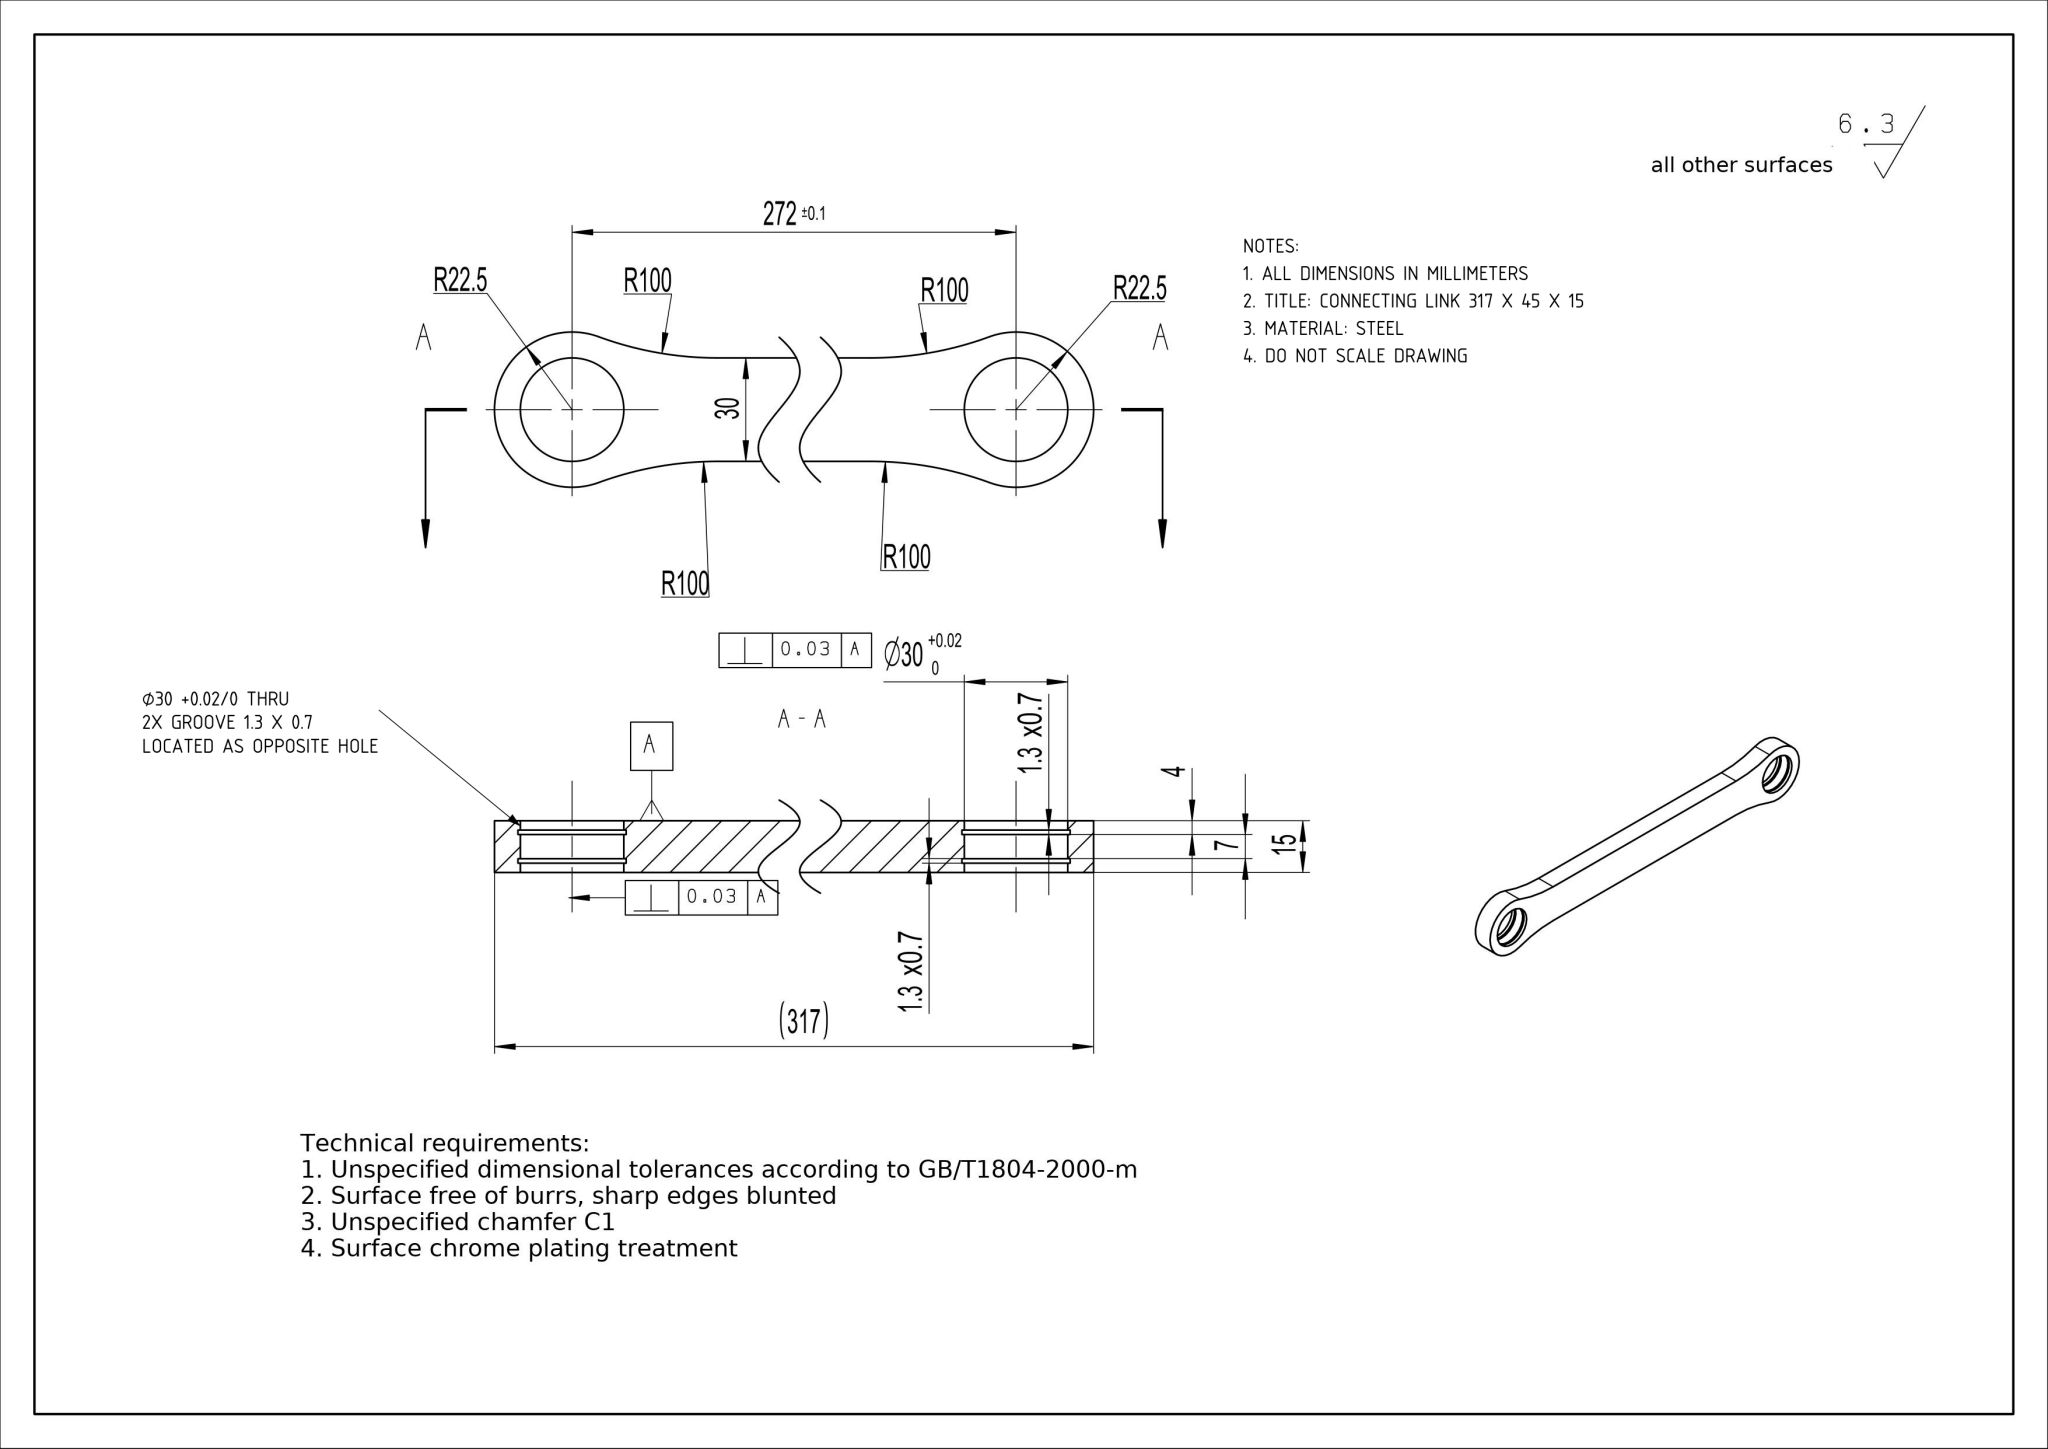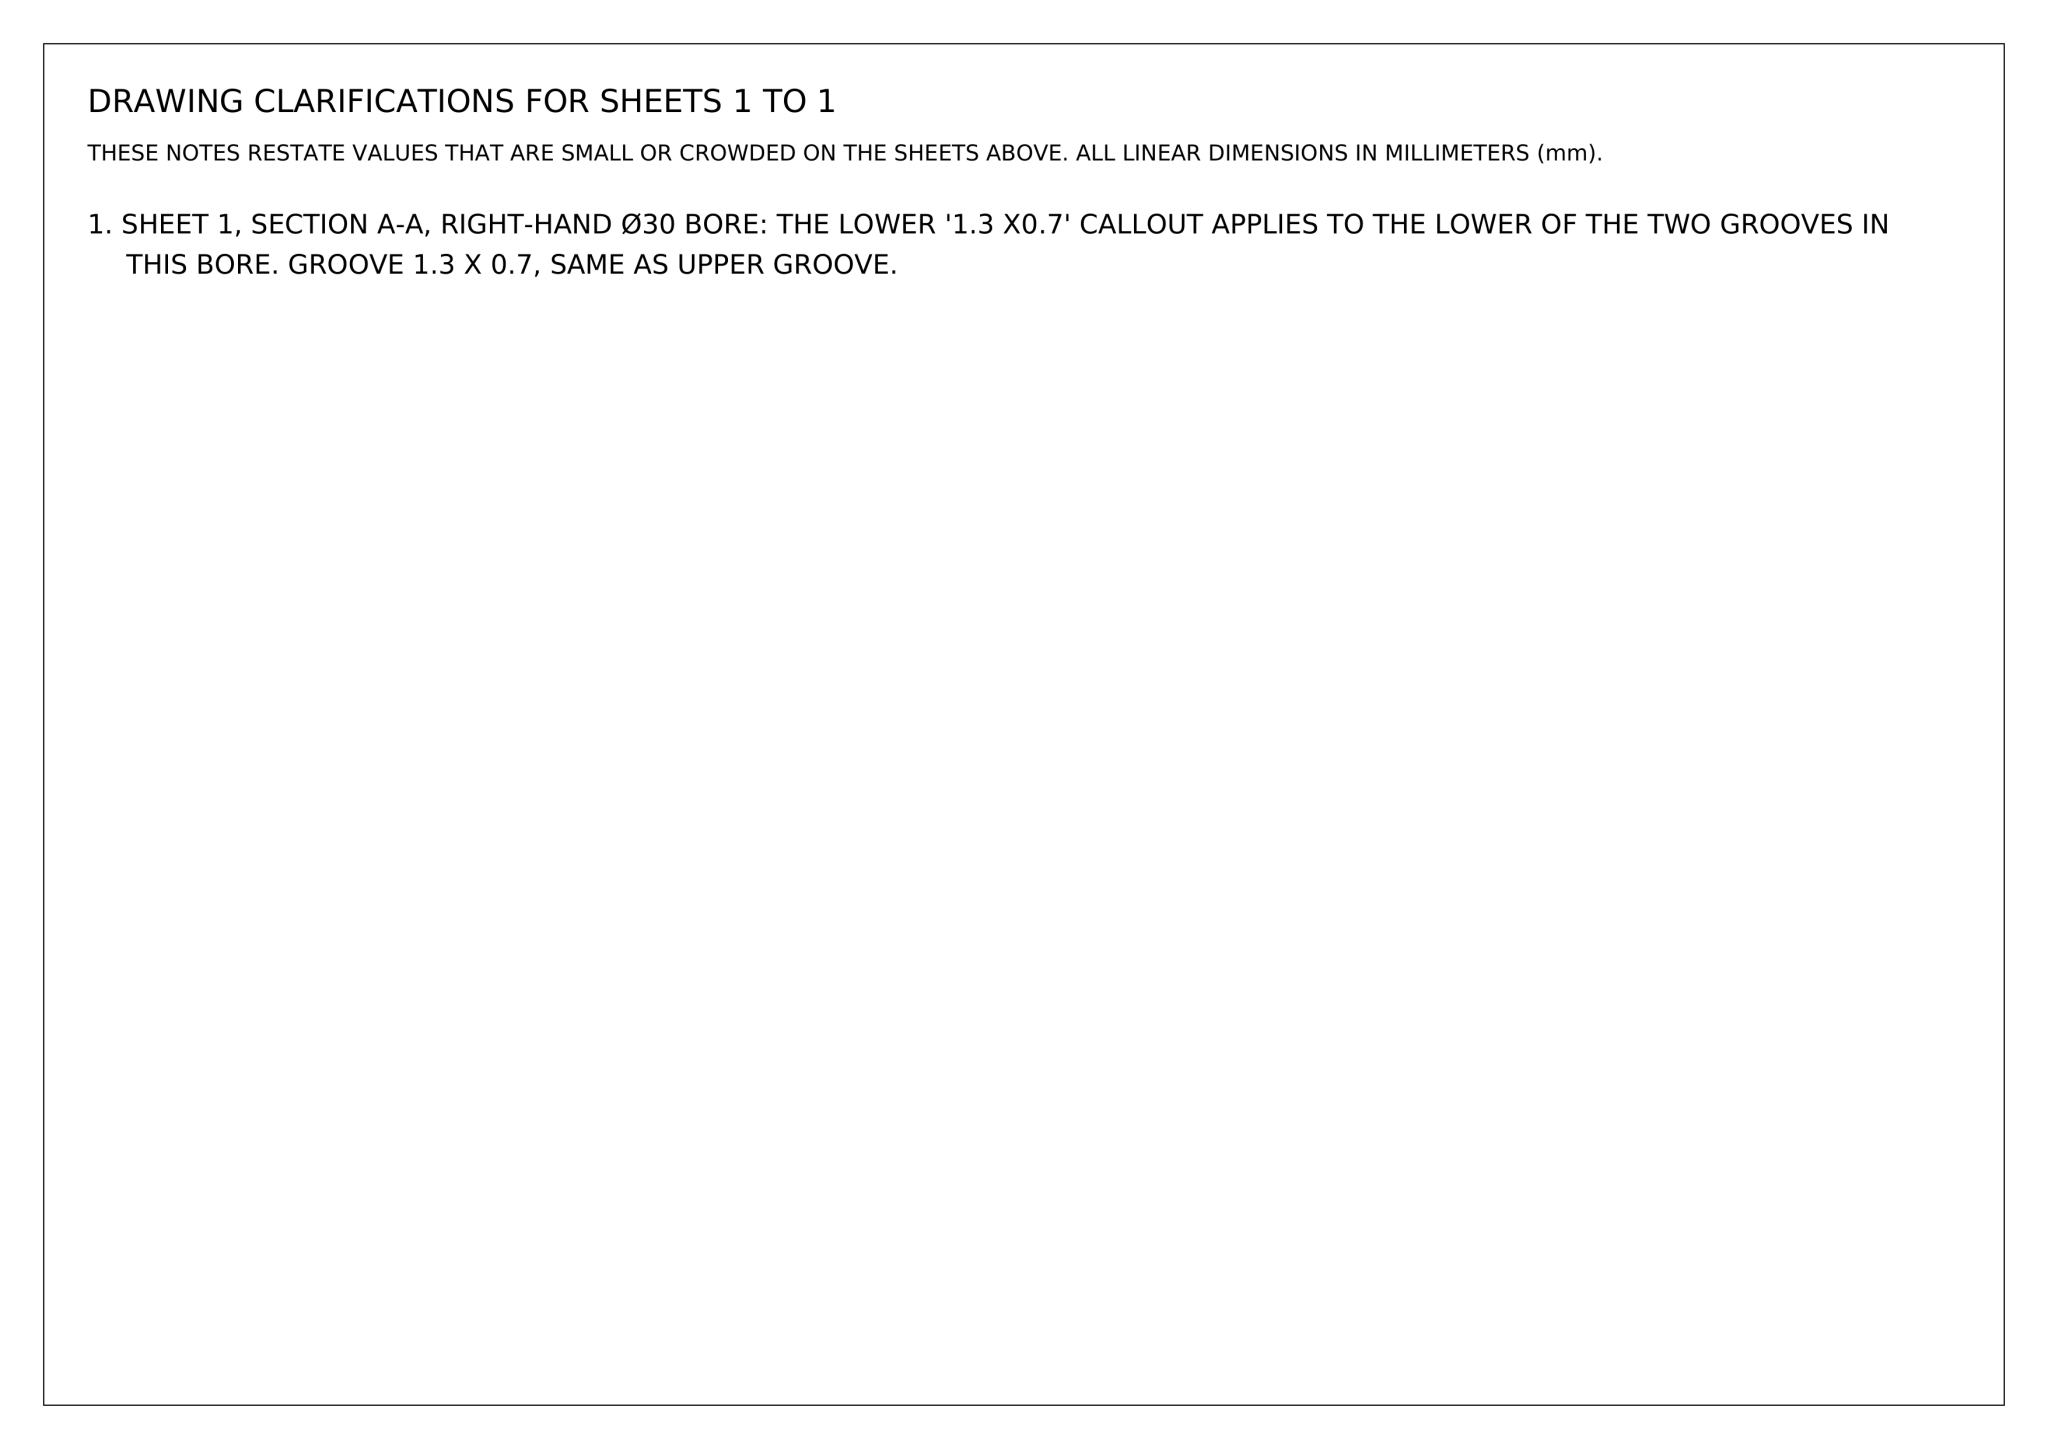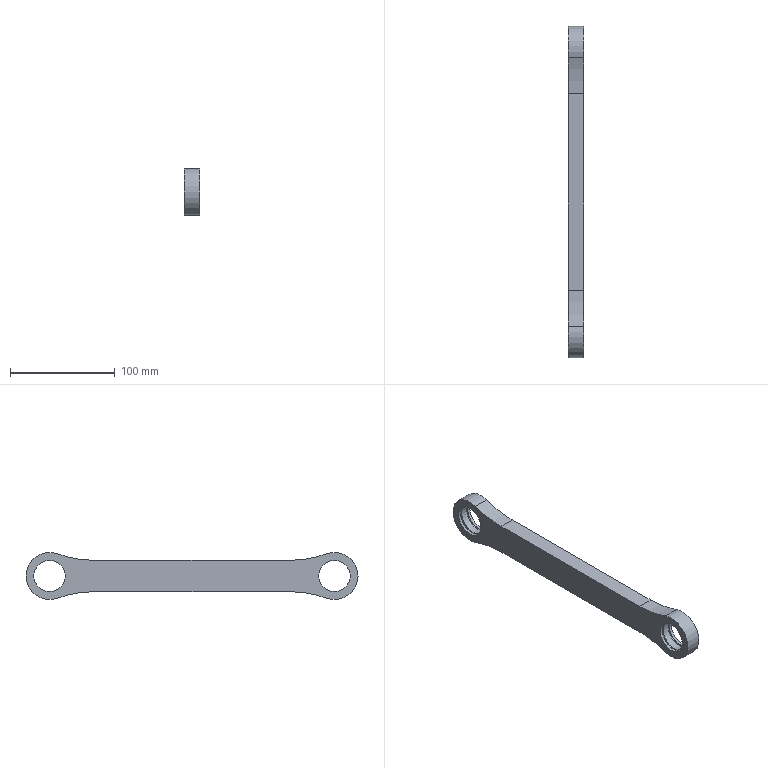Part | NX | mm | 1 solid | 28 faces | box 15 x 317 x 45 mm | volume 132143 mm3 | cylinder 16 | plane 12 | commonest cylinder face diameters 30 x6 31.4 x4 200 x4 45 x2
STEP:
#1=CARTESIAN_POINT('',(0.,0.,0.));
#2=DIRECTION('',(0.,0.,1.));
#3=DIRECTION('',(1.,0.,0.));
#4=AXIS2_PLACEMENT_3D('',#1,#2,#3);
#5=(LENGTH_UNIT()NAMED_UNIT(*)SI_UNIT(.MILLI.,.METRE.));
#6=UNCERTAINTY_MEASURE_WITH_UNIT(LENGTH_MEASURE(0.00002),#5,'','');
#7=(NAMED_UNIT(*)PLANE_ANGLE_UNIT()SI_UNIT($,.RADIAN.));
#8=PLANE_ANGLE_MEASURE_WITH_UNIT(PLANE_ANGLE_MEASURE(0.01745),#7);
#9=DIMENSIONAL_EXPONENTS(0.,0.,0.,0.,0.,0.,0.);
#10=(CONVERSION_BASED_UNIT('',#8)NAMED_UNIT(#9)PLANE_ANGLE_UNIT());
#11=(NAMED_UNIT(*)SI_UNIT($,.STERADIAN.)SOLID_ANGLE_UNIT());
#12=(GEOMETRIC_REPRESENTATION_CONTEXT(3)GLOBAL_UNCERTAINTY_ASSIGNED_CONTEXT((#6))GLOBAL_UNIT_ASSIGNED_CONTEXT((#5,#10,#11))REPRESENTATION_CONTEXT('',''));
#13=SHAPE_REPRESENTATION('',(#4),#12);
#14=CARTESIAN_POINT('',(4.,277.,-15.));
#15=VERTEX_POINT('',#14);
#16=CARTESIAN_POINT('',(4.,277.,0.));
#17=DIRECTION('',(1.,0.,0.));
#18=DIRECTION('',(0.,0.,-1.));
#19=AXIS2_PLACEMENT_3D('',#16,#17,#18);
#20=CIRCLE('',#19,15.);
#21=EDGE_CURVE('',#15,#15,#20,.T.);
#22=ORIENTED_EDGE('',*,*,#21,.F.);
#23=EDGE_LOOP('',(#22));
#24=FACE_BOUND('',#23,.T.);
#25=CARTESIAN_POINT('',(11.,277.,-15.));
#26=VERTEX_POINT('',#25);
#27=CARTESIAN_POINT('',(11.,277.,0.));
#28=DIRECTION('',(1.,0.,0.));
#29=DIRECTION('',(0.,0.,-1.));
#30=AXIS2_PLACEMENT_3D('',#27,#28,#29);
#31=CIRCLE('',#30,15.);
#32=EDGE_CURVE('',#26,#26,#31,.T.);
#33=ORIENTED_EDGE('',*,*,#32,.T.);
#34=EDGE_LOOP('',(#33));
#35=FACE_BOUND('',#34,.T.);
#36=CARTESIAN_POINT('',(15.,277.,0.));
#37=DIRECTION('',(-1.,0.,0.));
#38=DIRECTION('',(0.,0.,1.));
#39=AXIS2_PLACEMENT_3D('',#36,#37,#38);
#40=CYLINDRICAL_SURFACE('',#39,15.);
#41=ADVANCED_FACE('',(#24,#35),#40,.F.);
#42=CARTESIAN_POINT('',(0.,277.,-15.));
#43=VERTEX_POINT('',#42);
#44=CARTESIAN_POINT('',(0.,277.,0.));
#45=DIRECTION('',(1.,0.,0.));
#46=DIRECTION('',(0.,0.,-1.));
#47=AXIS2_PLACEMENT_3D('',#44,#45,#46);
#48=CIRCLE('',#47,15.);
#49=EDGE_CURVE('',#43,#43,#48,.T.);
#50=ORIENTED_EDGE('',*,*,#49,.F.);
#51=EDGE_LOOP('',(#50));
#52=FACE_BOUND('',#51,.T.);
#53=CARTESIAN_POINT('',(2.7,277.,-15.));
#54=VERTEX_POINT('',#53);
#55=CARTESIAN_POINT('',(2.7,277.,0.));
#56=DIRECTION('',(1.,0.,0.));
#57=DIRECTION('',(0.,0.,-1.));
#58=AXIS2_PLACEMENT_3D('',#55,#56,#57);
#59=CIRCLE('',#58,15.);
#60=EDGE_CURVE('',#54,#54,#59,.T.);
#61=ORIENTED_EDGE('',*,*,#60,.T.);
#62=EDGE_LOOP('',(#61));
#63=FACE_BOUND('',#62,.T.);
#64=CARTESIAN_POINT('',(15.,277.,0.));
#65=DIRECTION('',(-1.,0.,0.));
#66=DIRECTION('',(0.,0.,1.));
#67=AXIS2_PLACEMENT_3D('',#64,#65,#66);
#68=CYLINDRICAL_SURFACE('',#67,15.);
#69=ADVANCED_FACE('',(#52,#63),#68,.F.);
#70=CARTESIAN_POINT('',(4.,5.,-15.));
#71=VERTEX_POINT('',#70);
#72=CARTESIAN_POINT('',(4.,5.,0.));
#73=DIRECTION('',(1.,0.,0.));
#74=DIRECTION('',(0.,0.,-1.));
#75=AXIS2_PLACEMENT_3D('',#72,#73,#74);
#76=CIRCLE('',#75,15.);
#77=EDGE_CURVE('',#71,#71,#76,.T.);
#78=ORIENTED_EDGE('',*,*,#77,.F.);
#79=EDGE_LOOP('',(#78));
#80=FACE_BOUND('',#79,.T.);
#81=CARTESIAN_POINT('',(11.,5.,-15.));
#82=VERTEX_POINT('',#81);
#83=CARTESIAN_POINT('',(11.,5.,0.));
#84=DIRECTION('',(1.,0.,0.));
#85=DIRECTION('',(0.,0.,-1.));
#86=AXIS2_PLACEMENT_3D('',#83,#84,#85);
#87=CIRCLE('',#86,15.);
#88=EDGE_CURVE('',#82,#82,#87,.T.);
#89=ORIENTED_EDGE('',*,*,#88,.T.);
#90=EDGE_LOOP('',(#89));
#91=FACE_BOUND('',#90,.T.);
#92=CARTESIAN_POINT('',(15.,5.,0.));
#93=DIRECTION('',(-1.,0.,0.));
#94=DIRECTION('',(0.,0.,1.));
#95=AXIS2_PLACEMENT_3D('',#92,#93,#94);
#96=CYLINDRICAL_SURFACE('',#95,15.);
#97=ADVANCED_FACE('',(#80,#91),#96,.F.);
#98=CARTESIAN_POINT('',(0.,5.,-15.));
#99=VERTEX_POINT('',#98);
#100=CARTESIAN_POINT('',(0.,5.,0.));
#101=DIRECTION('',(1.,0.,0.));
#102=DIRECTION('',(0.,0.,-1.));
#103=AXIS2_PLACEMENT_3D('',#100,#101,#102);
#104=CIRCLE('',#103,15.);
#105=EDGE_CURVE('',#99,#99,#104,.T.);
#106=ORIENTED_EDGE('',*,*,#105,.F.);
#107=EDGE_LOOP('',(#106));
#108=FACE_BOUND('',#107,.T.);
#109=CARTESIAN_POINT('',(2.7,5.,-15.));
#110=VERTEX_POINT('',#109);
#111=CARTESIAN_POINT('',(2.7,5.,0.));
#112=DIRECTION('',(1.,0.,0.));
#113=DIRECTION('',(0.,0.,-1.));
#114=AXIS2_PLACEMENT_3D('',#111,#112,#113);
#115=CIRCLE('',#114,15.);
#116=EDGE_CURVE('',#110,#110,#115,.T.);
#117=ORIENTED_EDGE('',*,*,#116,.T.);
#118=EDGE_LOOP('',(#117));
#119=FACE_BOUND('',#118,.T.);
#120=CARTESIAN_POINT('',(15.,5.,0.));
#121=DIRECTION('',(-1.,0.,0.));
#122=DIRECTION('',(0.,0.,1.));
#123=AXIS2_PLACEMENT_3D('',#120,#121,#122);
#124=CYLINDRICAL_SURFACE('',#123,15.);
#125=ADVANCED_FACE('',(#108,#119),#124,.F.);
#126=CARTESIAN_POINT('',(0.,47.205,-15.));
#127=VERTEX_POINT('',#126);
#128=CARTESIAN_POINT('',(0.,234.795,-15.));
#129=VERTEX_POINT('',#128);
#130=CARTESIAN_POINT('',(0.,0.,-15.));
#131=DIRECTION('',(0.,1.,0.));
#132=VECTOR('',#131,1.);
#133=LINE('',#130,#132);
#134=EDGE_CURVE('',#127,#129,#133,.T.);
#135=ORIENTED_EDGE('',*,*,#134,.T.);
#136=CARTESIAN_POINT('',(15.,234.795,-15.));
#137=VERTEX_POINT('',#136);
#138=CARTESIAN_POINT('',(15.,234.795,-15.));
#139=DIRECTION('',(1.,0.,0.));
#140=VECTOR('',#139,1.);
#141=LINE('',#138,#140);
#142=EDGE_CURVE('',#129,#137,#141,.T.);
#143=ORIENTED_EDGE('',*,*,#142,.T.);
#144=CARTESIAN_POINT('',(15.,47.205,-15.));
#145=VERTEX_POINT('',#144);
#146=CARTESIAN_POINT('',(15.,0.,-15.));
#147=DIRECTION('',(0.,1.,0.));
#148=VECTOR('',#147,1.);
#149=LINE('',#146,#148);
#150=EDGE_CURVE('',#145,#137,#149,.T.);
#151=ORIENTED_EDGE('',*,*,#150,.F.);
#152=CARTESIAN_POINT('',(15.,47.205,-15.));
#153=DIRECTION('',(-1.,0.,0.));
#154=VECTOR('',#153,1.);
#155=LINE('',#152,#154);
#156=EDGE_CURVE('',#145,#127,#155,.T.);
#157=ORIENTED_EDGE('',*,*,#156,.T.);
#158=EDGE_LOOP('',(#135,#143,#151,#157));
#159=FACE_OUTER_BOUND('',#158,.T.);
#160=CARTESIAN_POINT('',(15.,0.,-15.));
#161=DIRECTION('',(0.,-0.,1.));
#162=DIRECTION('',(0.,-1.,-0.));
#163=AXIS2_PLACEMENT_3D('',#160,#161,#162);
#164=PLANE('',#163);
#165=ADVANCED_FACE('',(#159),#164,.F.);
#166=CARTESIAN_POINT('',(12.3,5.,-15.));
#167=VERTEX_POINT('',#166);
#168=CARTESIAN_POINT('',(12.3,5.,0.));
#169=DIRECTION('',(1.,0.,0.));
#170=DIRECTION('',(0.,0.,-1.));
#171=AXIS2_PLACEMENT_3D('',#168,#169,#170);
#172=CIRCLE('',#171,15.);
#173=EDGE_CURVE('',#167,#167,#172,.T.);
#174=ORIENTED_EDGE('',*,*,#173,.F.);
#175=EDGE_LOOP('',(#174));
#176=FACE_BOUND('',#175,.T.);
#177=CARTESIAN_POINT('',(15.,5.,-15.));
#178=VERTEX_POINT('',#177);
#179=CARTESIAN_POINT('',(15.,5.,0.));
#180=DIRECTION('',(1.,0.,0.));
#181=DIRECTION('',(0.,0.,-1.));
#182=AXIS2_PLACEMENT_3D('',#179,#180,#181);
#183=CIRCLE('',#182,15.);
#184=EDGE_CURVE('',#178,#178,#183,.T.);
#185=ORIENTED_EDGE('',*,*,#184,.T.);
#186=EDGE_LOOP('',(#185));
#187=FACE_BOUND('',#186,.T.);
#188=CARTESIAN_POINT('',(15.,5.,0.));
#189=DIRECTION('',(-1.,0.,0.));
#190=DIRECTION('',(0.,0.,1.));
#191=AXIS2_PLACEMENT_3D('',#188,#189,#190);
#192=CYLINDRICAL_SURFACE('',#191,15.);
#193=ADVANCED_FACE('',(#176,#187),#192,.F.);
#194=CARTESIAN_POINT('',(15.,234.795,15.));
#195=VERTEX_POINT('',#194);
#196=CARTESIAN_POINT('',(15.,47.205,15.));
#197=VERTEX_POINT('',#196);
#198=CARTESIAN_POINT('',(15.,277.,15.));
#199=DIRECTION('',(0.,-1.,0.));
#200=VECTOR('',#199,1.);
#201=LINE('',#198,#200);
#202=EDGE_CURVE('',#195,#197,#201,.T.);
#203=ORIENTED_EDGE('',*,*,#202,.F.);
#204=CARTESIAN_POINT('',(0.,234.795,15.));
#205=VERTEX_POINT('',#204);
#206=CARTESIAN_POINT('',(15.,234.795,15.));
#207=DIRECTION('',(-1.,0.,0.));
#208=VECTOR('',#207,1.);
#209=LINE('',#206,#208);
#210=EDGE_CURVE('',#195,#205,#209,.T.);
#211=ORIENTED_EDGE('',*,*,#210,.T.);
#212=CARTESIAN_POINT('',(0.,47.205,15.));
#213=VERTEX_POINT('',#212);
#214=CARTESIAN_POINT('',(0.,277.,15.));
#215=DIRECTION('',(0.,-1.,0.));
#216=VECTOR('',#215,1.);
#217=LINE('',#214,#216);
#218=EDGE_CURVE('',#205,#213,#217,.T.);
#219=ORIENTED_EDGE('',*,*,#218,.T.);
#220=CARTESIAN_POINT('',(15.,47.205,15.));
#221=DIRECTION('',(1.,0.,0.));
#222=VECTOR('',#221,1.);
#223=LINE('',#220,#222);
#224=EDGE_CURVE('',#213,#197,#223,.T.);
#225=ORIENTED_EDGE('',*,*,#224,.T.);
#226=EDGE_LOOP('',(#203,#211,#219,#225));
#227=FACE_OUTER_BOUND('',#226,.T.);
#228=CARTESIAN_POINT('',(15.,277.,15.));
#229=DIRECTION('',(0.,0.,-1.));
#230=DIRECTION('',(-1.,0.,0.));
#231=AXIS2_PLACEMENT_3D('',#228,#229,#230);
#232=PLANE('',#231);
#233=ADVANCED_FACE('',(#227),#232,.F.);
#234=CARTESIAN_POINT('',(12.3,277.,-15.));
#235=VERTEX_POINT('',#234);
#236=CARTESIAN_POINT('',(12.3,277.,0.));
#237=DIRECTION('',(1.,0.,0.));
#238=DIRECTION('',(0.,0.,-1.));
#239=AXIS2_PLACEMENT_3D('',#236,#237,#238);
#240=CIRCLE('',#239,15.);
#241=EDGE_CURVE('',#235,#235,#240,.T.);
#242=ORIENTED_EDGE('',*,*,#241,.F.);
#243=EDGE_LOOP('',(#242));
#244=FACE_BOUND('',#243,.T.);
#245=CARTESIAN_POINT('',(15.,277.,-15.));
#246=VERTEX_POINT('',#245);
#247=CARTESIAN_POINT('',(15.,277.,0.));
#248=DIRECTION('',(1.,0.,0.));
#249=DIRECTION('',(0.,0.,-1.));
#250=AXIS2_PLACEMENT_3D('',#247,#248,#249);
#251=CIRCLE('',#250,15.);
#252=EDGE_CURVE('',#246,#246,#251,.T.);
#253=ORIENTED_EDGE('',*,*,#252,.T.);
#254=EDGE_LOOP('',(#253));
#255=FACE_BOUND('',#254,.T.);
#256=CARTESIAN_POINT('',(15.,277.,0.));
#257=DIRECTION('',(-1.,0.,0.));
#258=DIRECTION('',(0.,0.,1.));
#259=AXIS2_PLACEMENT_3D('',#256,#257,#258);
#260=CYLINDRICAL_SURFACE('',#259,15.);
#261=ADVANCED_FACE('',(#244,#255),#260,.F.);
#262=ORIENTED_EDGE('',*,*,#150,.T.);
#263=CARTESIAN_POINT('',(15.,269.248,-21.122));
#264=VERTEX_POINT('',#263);
#265=CARTESIAN_POINT('',(15.,234.795,-115.));
#266=DIRECTION('',(-1.,0.,0.));
#267=DIRECTION('',(0.,0.,-1.));
#268=AXIS2_PLACEMENT_3D('',#265,#266,#267);
#269=CIRCLE('',#268,100.);
#270=EDGE_CURVE('',#137,#264,#269,.T.);
#271=ORIENTED_EDGE('',*,*,#270,.T.);
#272=CARTESIAN_POINT('',(15.,269.248,21.122));
#273=VERTEX_POINT('',#272);
#274=CARTESIAN_POINT('',(15.,277.,0.));
#275=DIRECTION('',(1.,0.,0.));
#276=DIRECTION('',(0.,-1.,0.));
#277=AXIS2_PLACEMENT_3D('',#274,#275,#276);
#278=CIRCLE('',#277,22.5);
#279=EDGE_CURVE('',#264,#273,#278,.T.);
#280=ORIENTED_EDGE('',*,*,#279,.T.);
#281=CARTESIAN_POINT('',(15.,234.795,115.));
#282=DIRECTION('',(-1.,0.,0.));
#283=DIRECTION('',(0.,0.,-1.));
#284=AXIS2_PLACEMENT_3D('',#281,#282,#283);
#285=CIRCLE('',#284,100.);
#286=EDGE_CURVE('',#273,#195,#285,.T.);
#287=ORIENTED_EDGE('',*,*,#286,.T.);
#288=ORIENTED_EDGE('',*,*,#202,.T.);
#289=CARTESIAN_POINT('',(15.,12.752,21.122));
#290=VERTEX_POINT('',#289);
#291=CARTESIAN_POINT('',(15.,47.205,115.));
#292=DIRECTION('',(-1.,0.,0.));
#293=DIRECTION('',(0.,0.,-1.));
#294=AXIS2_PLACEMENT_3D('',#291,#292,#293);
#295=CIRCLE('',#294,100.);
#296=EDGE_CURVE('',#197,#290,#295,.T.);
#297=ORIENTED_EDGE('',*,*,#296,.T.);
#298=CARTESIAN_POINT('',(15.,12.752,-21.122));
#299=VERTEX_POINT('',#298);
#300=CARTESIAN_POINT('',(15.,5.,0.));
#301=DIRECTION('',(1.,0.,0.));
#302=DIRECTION('',(0.,1.,-0.));
#303=AXIS2_PLACEMENT_3D('',#300,#301,#302);
#304=CIRCLE('',#303,22.5);
#305=EDGE_CURVE('',#290,#299,#304,.T.);
#306=ORIENTED_EDGE('',*,*,#305,.T.);
#307=CARTESIAN_POINT('',(15.,47.205,-115.));
#308=DIRECTION('',(-1.,0.,0.));
#309=DIRECTION('',(0.,0.,-1.));
#310=AXIS2_PLACEMENT_3D('',#307,#308,#309);
#311=CIRCLE('',#310,100.);
#312=EDGE_CURVE('',#299,#145,#311,.T.);
#313=ORIENTED_EDGE('',*,*,#312,.T.);
#314=EDGE_LOOP('',(#262,#271,#280,#287,#288,#297,#306,#313));
#315=FACE_BOUND('',#314,.T.);
#316=ORIENTED_EDGE('',*,*,#184,.F.);
#317=EDGE_LOOP('',(#316));
#318=FACE_BOUND('',#317,.T.);
#319=ORIENTED_EDGE('',*,*,#252,.F.);
#320=EDGE_LOOP('',(#319));
#321=FACE_BOUND('',#320,.T.);
#322=CARTESIAN_POINT('',(15.,0.,0.));
#323=DIRECTION('',(1.,0.,0.));
#324=DIRECTION('',(0.,0.,-1.));
#325=AXIS2_PLACEMENT_3D('',#322,#323,#324);
#326=PLANE('',#325);
#327=ADVANCED_FACE('',(#315,#318,#321),#326,.T.);
#328=ORIENTED_EDGE('',*,*,#218,.F.);
#329=CARTESIAN_POINT('',(0.,269.248,21.122));
#330=VERTEX_POINT('',#329);
#331=CARTESIAN_POINT('',(0.,234.795,115.));
#332=DIRECTION('',(1.,0.,0.));
#333=DIRECTION('',(0.,0.,-1.));
#334=AXIS2_PLACEMENT_3D('',#331,#332,#333);
#335=CIRCLE('',#334,100.);
#336=EDGE_CURVE('',#205,#330,#335,.T.);
#337=ORIENTED_EDGE('',*,*,#336,.T.);
#338=CARTESIAN_POINT('',(0.,269.248,-21.122));
#339=VERTEX_POINT('',#338);
#340=CARTESIAN_POINT('',(0.,277.,0.));
#341=DIRECTION('',(1.,0.,0.));
#342=DIRECTION('',(0.,-1.,0.));
#343=AXIS2_PLACEMENT_3D('',#340,#341,#342);
#344=CIRCLE('',#343,22.5);
#345=EDGE_CURVE('',#339,#330,#344,.T.);
#346=ORIENTED_EDGE('',*,*,#345,.F.);
#347=CARTESIAN_POINT('',(0.,234.795,-115.));
#348=DIRECTION('',(1.,0.,0.));
#349=DIRECTION('',(0.,0.,-1.));
#350=AXIS2_PLACEMENT_3D('',#347,#348,#349);
#351=CIRCLE('',#350,100.);
#352=EDGE_CURVE('',#339,#129,#351,.T.);
#353=ORIENTED_EDGE('',*,*,#352,.T.);
#354=ORIENTED_EDGE('',*,*,#134,.F.);
#355=CARTESIAN_POINT('',(0.,12.752,-21.122));
#356=VERTEX_POINT('',#355);
#357=CARTESIAN_POINT('',(0.,47.205,-115.));
#358=DIRECTION('',(1.,0.,0.));
#359=DIRECTION('',(0.,0.,-1.));
#360=AXIS2_PLACEMENT_3D('',#357,#358,#359);
#361=CIRCLE('',#360,100.);
#362=EDGE_CURVE('',#127,#356,#361,.T.);
#363=ORIENTED_EDGE('',*,*,#362,.T.);
#364=CARTESIAN_POINT('',(0.,12.752,21.122));
#365=VERTEX_POINT('',#364);
#366=CARTESIAN_POINT('',(0.,5.,0.));
#367=DIRECTION('',(1.,0.,0.));
#368=DIRECTION('',(0.,1.,-0.));
#369=AXIS2_PLACEMENT_3D('',#366,#367,#368);
#370=CIRCLE('',#369,22.5);
#371=EDGE_CURVE('',#365,#356,#370,.T.);
#372=ORIENTED_EDGE('',*,*,#371,.F.);
#373=CARTESIAN_POINT('',(0.,47.205,115.));
#374=DIRECTION('',(1.,0.,0.));
#375=DIRECTION('',(0.,0.,-1.));
#376=AXIS2_PLACEMENT_3D('',#373,#374,#375);
#377=CIRCLE('',#376,100.);
#378=EDGE_CURVE('',#365,#213,#377,.T.);
#379=ORIENTED_EDGE('',*,*,#378,.T.);
#380=EDGE_LOOP('',(#328,#337,#346,#353,#354,#363,#372,#379));
#381=FACE_BOUND('',#380,.T.);
#382=ORIENTED_EDGE('',*,*,#105,.T.);
#383=EDGE_LOOP('',(#382));
#384=FACE_BOUND('',#383,.T.);
#385=ORIENTED_EDGE('',*,*,#49,.T.);
#386=EDGE_LOOP('',(#385));
#387=FACE_BOUND('',#386,.T.);
#388=CARTESIAN_POINT('',(0.,0.,0.));
#389=DIRECTION('',(1.,0.,0.));
#390=DIRECTION('',(0.,0.,-1.));
#391=AXIS2_PLACEMENT_3D('',#388,#389,#390);
#392=PLANE('',#391);
#393=ADVANCED_FACE('',(#381,#384,#387),#392,.F.);
#394=ORIENTED_EDGE('',*,*,#371,.T.);
#395=CARTESIAN_POINT('',(0.,12.752,-21.122));
#396=DIRECTION('',(1.,0.,0.));
#397=VECTOR('',#396,1.);
#398=LINE('',#395,#397);
#399=EDGE_CURVE('',#356,#299,#398,.T.);
#400=ORIENTED_EDGE('',*,*,#399,.T.);
#401=ORIENTED_EDGE('',*,*,#305,.F.);
#402=CARTESIAN_POINT('',(15.,12.752,21.122));
#403=DIRECTION('',(-1.,0.,0.));
#404=VECTOR('',#403,1.);
#405=LINE('',#402,#404);
#406=EDGE_CURVE('',#290,#365,#405,.T.);
#407=ORIENTED_EDGE('',*,*,#406,.T.);
#408=EDGE_LOOP('',(#394,#400,#401,#407));
#409=FACE_OUTER_BOUND('',#408,.T.);
#410=CARTESIAN_POINT('',(0.,5.,0.));
#411=DIRECTION('',(1.,0.,0.));
#412=DIRECTION('',(0.,0.,-1.));
#413=AXIS2_PLACEMENT_3D('',#410,#411,#412);
#414=CYLINDRICAL_SURFACE('',#413,22.5);
#415=ADVANCED_FACE('',(#409),#414,.T.);
#416=CARTESIAN_POINT('',(4.,5.,-15.7));
#417=VERTEX_POINT('',#416);
#418=CARTESIAN_POINT('',(4.,5.,0.));
#419=DIRECTION('',(-1.,0.,0.));
#420=DIRECTION('',(0.,0.,-1.));
#421=AXIS2_PLACEMENT_3D('',#418,#419,#420);
#422=CIRCLE('',#421,15.7);
#423=EDGE_CURVE('',#417,#417,#422,.T.);
#424=ORIENTED_EDGE('',*,*,#423,.F.);
#425=EDGE_LOOP('',(#424));
#426=FACE_BOUND('',#425,.T.);
#427=CARTESIAN_POINT('',(2.7,5.,-15.7));
#428=VERTEX_POINT('',#427);
#429=CARTESIAN_POINT('',(2.7,5.,0.));
#430=DIRECTION('',(-1.,0.,0.));
#431=DIRECTION('',(0.,0.,-1.));
#432=AXIS2_PLACEMENT_3D('',#429,#430,#431);
#433=CIRCLE('',#432,15.7);
#434=EDGE_CURVE('',#428,#428,#433,.T.);
#435=ORIENTED_EDGE('',*,*,#434,.T.);
#436=EDGE_LOOP('',(#435));
#437=FACE_BOUND('',#436,.T.);
#438=CARTESIAN_POINT('',(3.35,5.,0.));
#439=DIRECTION('',(1.,0.,0.));
#440=DIRECTION('',(0.,0.,-1.));
#441=AXIS2_PLACEMENT_3D('',#438,#439,#440);
#442=CYLINDRICAL_SURFACE('',#441,15.7);
#443=ADVANCED_FACE('',(#426,#437),#442,.F.);
#444=ORIENTED_EDGE('',*,*,#116,.F.);
#445=EDGE_LOOP('',(#444));
#446=FACE_BOUND('',#445,.T.);
#447=ORIENTED_EDGE('',*,*,#434,.F.);
#448=EDGE_LOOP('',(#447));
#449=FACE_BOUND('',#448,.T.);
#450=CARTESIAN_POINT('',(2.7,0.,0.));
#451=DIRECTION('',(1.,0.,0.));
#452=DIRECTION('',(0.,0.,-1.));
#453=AXIS2_PLACEMENT_3D('',#450,#451,#452);
#454=PLANE('',#453);
#455=ADVANCED_FACE('',(#446,#449),#454,.T.);
#456=ORIENTED_EDGE('',*,*,#77,.T.);
#457=EDGE_LOOP('',(#456));
#458=FACE_BOUND('',#457,.T.);
#459=ORIENTED_EDGE('',*,*,#423,.T.);
#460=EDGE_LOOP('',(#459));
#461=FACE_BOUND('',#460,.T.);
#462=CARTESIAN_POINT('',(4.,0.,0.));
#463=DIRECTION('',(1.,0.,0.));
#464=DIRECTION('',(0.,0.,-1.));
#465=AXIS2_PLACEMENT_3D('',#462,#463,#464);
#466=PLANE('',#465);
#467=ADVANCED_FACE('',(#458,#461),#466,.F.);
#468=CARTESIAN_POINT('',(12.3,5.,-15.7));
#469=VERTEX_POINT('',#468);
#470=CARTESIAN_POINT('',(12.3,5.,0.));
#471=DIRECTION('',(-1.,0.,0.));
#472=DIRECTION('',(0.,0.,-1.));
#473=AXIS2_PLACEMENT_3D('',#470,#471,#472);
#474=CIRCLE('',#473,15.7);
#475=EDGE_CURVE('',#469,#469,#474,.T.);
#476=ORIENTED_EDGE('',*,*,#475,.F.);
#477=EDGE_LOOP('',(#476));
#478=FACE_BOUND('',#477,.T.);
#479=CARTESIAN_POINT('',(11.,5.,-15.7));
#480=VERTEX_POINT('',#479);
#481=CARTESIAN_POINT('',(11.,5.,0.));
#482=DIRECTION('',(-1.,0.,0.));
#483=DIRECTION('',(0.,0.,-1.));
#484=AXIS2_PLACEMENT_3D('',#481,#482,#483);
#485=CIRCLE('',#484,15.7);
#486=EDGE_CURVE('',#480,#480,#485,.T.);
#487=ORIENTED_EDGE('',*,*,#486,.T.);
#488=EDGE_LOOP('',(#487));
#489=FACE_BOUND('',#488,.T.);
#490=CARTESIAN_POINT('',(11.65,5.,0.));
#491=DIRECTION('',(1.,0.,0.));
#492=DIRECTION('',(0.,0.,-1.));
#493=AXIS2_PLACEMENT_3D('',#490,#491,#492);
#494=CYLINDRICAL_SURFACE('',#493,15.7);
#495=ADVANCED_FACE('',(#478,#489),#494,.F.);
#496=ORIENTED_EDGE('',*,*,#88,.F.);
#497=EDGE_LOOP('',(#496));
#498=FACE_BOUND('',#497,.T.);
#499=ORIENTED_EDGE('',*,*,#486,.F.);
#500=EDGE_LOOP('',(#499));
#501=FACE_BOUND('',#500,.T.);
#502=CARTESIAN_POINT('',(11.,0.,0.));
#503=DIRECTION('',(1.,0.,0.));
#504=DIRECTION('',(0.,0.,-1.));
#505=AXIS2_PLACEMENT_3D('',#502,#503,#504);
#506=PLANE('',#505);
#507=ADVANCED_FACE('',(#498,#501),#506,.T.);
#508=ORIENTED_EDGE('',*,*,#173,.T.);
#509=EDGE_LOOP('',(#508));
#510=FACE_BOUND('',#509,.T.);
#511=ORIENTED_EDGE('',*,*,#475,.T.);
#512=EDGE_LOOP('',(#511));
#513=FACE_BOUND('',#512,.T.);
#514=CARTESIAN_POINT('',(12.3,0.,0.));
#515=DIRECTION('',(1.,0.,0.));
#516=DIRECTION('',(0.,0.,-1.));
#517=AXIS2_PLACEMENT_3D('',#514,#515,#516);
#518=PLANE('',#517);
#519=ADVANCED_FACE('',(#510,#513),#518,.F.);
#520=ORIENTED_EDGE('',*,*,#345,.T.);
#521=CARTESIAN_POINT('',(0.,269.248,21.122));
#522=DIRECTION('',(1.,0.,0.));
#523=VECTOR('',#522,1.);
#524=LINE('',#521,#523);
#525=EDGE_CURVE('',#330,#273,#524,.T.);
#526=ORIENTED_EDGE('',*,*,#525,.T.);
#527=ORIENTED_EDGE('',*,*,#279,.F.);
#528=CARTESIAN_POINT('',(0.,269.248,-21.122));
#529=DIRECTION('',(-1.,0.,0.));
#530=VECTOR('',#529,1.);
#531=LINE('',#528,#530);
#532=EDGE_CURVE('',#264,#339,#531,.T.);
#533=ORIENTED_EDGE('',*,*,#532,.T.);
#534=EDGE_LOOP('',(#520,#526,#527,#533));
#535=FACE_OUTER_BOUND('',#534,.T.);
#536=CARTESIAN_POINT('',(0.,277.,0.));
#537=DIRECTION('',(1.,0.,0.));
#538=DIRECTION('',(0.,0.,-1.));
#539=AXIS2_PLACEMENT_3D('',#536,#537,#538);
#540=CYLINDRICAL_SURFACE('',#539,22.5);
#541=ADVANCED_FACE('',(#535),#540,.T.);
#542=ORIENTED_EDGE('',*,*,#286,.F.);
#543=ORIENTED_EDGE('',*,*,#525,.F.);
#544=ORIENTED_EDGE('',*,*,#336,.F.);
#545=ORIENTED_EDGE('',*,*,#210,.F.);
#546=EDGE_LOOP('',(#542,#543,#544,#545));
#547=FACE_OUTER_BOUND('',#546,.T.);
#548=CARTESIAN_POINT('',(0.,234.795,115.));
#549=DIRECTION('',(1.,0.,0.));
#550=DIRECTION('',(0.,0.,-1.));
#551=AXIS2_PLACEMENT_3D('',#548,#549,#550);
#552=CYLINDRICAL_SURFACE('',#551,100.);
#553=ADVANCED_FACE('',(#547),#552,.F.);
#554=ORIENTED_EDGE('',*,*,#352,.F.);
#555=ORIENTED_EDGE('',*,*,#532,.F.);
#556=ORIENTED_EDGE('',*,*,#270,.F.);
#557=ORIENTED_EDGE('',*,*,#142,.F.);
#558=EDGE_LOOP('',(#554,#555,#556,#557));
#559=FACE_OUTER_BOUND('',#558,.T.);
#560=CARTESIAN_POINT('',(0.,234.795,-115.));
#561=DIRECTION('',(1.,0.,0.));
#562=DIRECTION('',(0.,0.,-1.));
#563=AXIS2_PLACEMENT_3D('',#560,#561,#562);
#564=CYLINDRICAL_SURFACE('',#563,100.);
#565=ADVANCED_FACE('',(#559),#564,.F.);
#566=ORIENTED_EDGE('',*,*,#312,.F.);
#567=ORIENTED_EDGE('',*,*,#399,.F.);
#568=ORIENTED_EDGE('',*,*,#362,.F.);
#569=ORIENTED_EDGE('',*,*,#156,.F.);
#570=EDGE_LOOP('',(#566,#567,#568,#569));
#571=FACE_OUTER_BOUND('',#570,.T.);
#572=CARTESIAN_POINT('',(0.,47.205,-115.));
#573=DIRECTION('',(1.,0.,0.));
#574=DIRECTION('',(0.,0.,-1.));
#575=AXIS2_PLACEMENT_3D('',#572,#573,#574);
#576=CYLINDRICAL_SURFACE('',#575,100.);
#577=ADVANCED_FACE('',(#571),#576,.F.);
#578=ORIENTED_EDGE('',*,*,#378,.F.);
#579=ORIENTED_EDGE('',*,*,#406,.F.);
#580=ORIENTED_EDGE('',*,*,#296,.F.);
#581=ORIENTED_EDGE('',*,*,#224,.F.);
#582=EDGE_LOOP('',(#578,#579,#580,#581));
#583=FACE_OUTER_BOUND('',#582,.T.);
#584=CARTESIAN_POINT('',(0.,47.205,115.));
#585=DIRECTION('',(1.,0.,0.));
#586=DIRECTION('',(0.,0.,-1.));
#587=AXIS2_PLACEMENT_3D('',#584,#585,#586);
#588=CYLINDRICAL_SURFACE('',#587,100.);
#589=ADVANCED_FACE('',(#583),#588,.F.);
#590=CARTESIAN_POINT('',(4.,277.,-15.7));
#591=VERTEX_POINT('',#590);
#592=CARTESIAN_POINT('',(4.,277.,0.));
#593=DIRECTION('',(-1.,0.,0.));
#594=DIRECTION('',(0.,0.,-1.));
#595=AXIS2_PLACEMENT_3D('',#592,#593,#594);
#596=CIRCLE('',#595,15.7);
#597=EDGE_CURVE('',#591,#591,#596,.T.);
#598=ORIENTED_EDGE('',*,*,#597,.F.);
#599=EDGE_LOOP('',(#598));
#600=FACE_BOUND('',#599,.T.);
#601=CARTESIAN_POINT('',(2.7,277.,-15.7));
#602=VERTEX_POINT('',#601);
#603=CARTESIAN_POINT('',(2.7,277.,0.));
#604=DIRECTION('',(-1.,0.,0.));
#605=DIRECTION('',(0.,0.,-1.));
#606=AXIS2_PLACEMENT_3D('',#603,#604,#605);
#607=CIRCLE('',#606,15.7);
#608=EDGE_CURVE('',#602,#602,#607,.T.);
#609=ORIENTED_EDGE('',*,*,#608,.T.);
#610=EDGE_LOOP('',(#609));
#611=FACE_BOUND('',#610,.T.);
#612=CARTESIAN_POINT('',(3.35,277.,0.));
#613=DIRECTION('',(1.,0.,0.));
#614=DIRECTION('',(0.,0.,-1.));
#615=AXIS2_PLACEMENT_3D('',#612,#613,#614);
#616=CYLINDRICAL_SURFACE('',#615,15.7);
#617=ADVANCED_FACE('',(#600,#611),#616,.F.);
#618=ORIENTED_EDGE('',*,*,#60,.F.);
#619=EDGE_LOOP('',(#618));
#620=FACE_BOUND('',#619,.T.);
#621=ORIENTED_EDGE('',*,*,#608,.F.);
#622=EDGE_LOOP('',(#621));
#623=FACE_BOUND('',#622,.T.);
#624=CARTESIAN_POINT('',(2.7,277.,0.));
#625=DIRECTION('',(1.,0.,0.));
#626=DIRECTION('',(0.,0.,-1.));
#627=AXIS2_PLACEMENT_3D('',#624,#625,#626);
#628=PLANE('',#627);
#629=ADVANCED_FACE('',(#620,#623),#628,.T.);
#630=ORIENTED_EDGE('',*,*,#21,.T.);
#631=EDGE_LOOP('',(#630));
#632=FACE_BOUND('',#631,.T.);
#633=ORIENTED_EDGE('',*,*,#597,.T.);
#634=EDGE_LOOP('',(#633));
#635=FACE_BOUND('',#634,.T.);
#636=CARTESIAN_POINT('',(4.,277.,0.));
#637=DIRECTION('',(1.,0.,0.));
#638=DIRECTION('',(0.,0.,-1.));
#639=AXIS2_PLACEMENT_3D('',#636,#637,#638);
#640=PLANE('',#639);
#641=ADVANCED_FACE('',(#632,#635),#640,.F.);
#642=CARTESIAN_POINT('',(12.3,277.,-15.7));
#643=VERTEX_POINT('',#642);
#644=CARTESIAN_POINT('',(12.3,277.,0.));
#645=DIRECTION('',(-1.,0.,0.));
#646=DIRECTION('',(0.,0.,-1.));
#647=AXIS2_PLACEMENT_3D('',#644,#645,#646);
#648=CIRCLE('',#647,15.7);
#649=EDGE_CURVE('',#643,#643,#648,.T.);
#650=ORIENTED_EDGE('',*,*,#649,.F.);
#651=EDGE_LOOP('',(#650));
#652=FACE_BOUND('',#651,.T.);
#653=CARTESIAN_POINT('',(11.,277.,-15.7));
#654=VERTEX_POINT('',#653);
#655=CARTESIAN_POINT('',(11.,277.,0.));
#656=DIRECTION('',(-1.,0.,0.));
#657=DIRECTION('',(0.,0.,-1.));
#658=AXIS2_PLACEMENT_3D('',#655,#656,#657);
#659=CIRCLE('',#658,15.7);
#660=EDGE_CURVE('',#654,#654,#659,.T.);
#661=ORIENTED_EDGE('',*,*,#660,.T.);
#662=EDGE_LOOP('',(#661));
#663=FACE_BOUND('',#662,.T.);
#664=CARTESIAN_POINT('',(11.65,277.,0.));
#665=DIRECTION('',(1.,0.,0.));
#666=DIRECTION('',(0.,0.,-1.));
#667=AXIS2_PLACEMENT_3D('',#664,#665,#666);
#668=CYLINDRICAL_SURFACE('',#667,15.7);
#669=ADVANCED_FACE('',(#652,#663),#668,.F.);
#670=ORIENTED_EDGE('',*,*,#32,.F.);
#671=EDGE_LOOP('',(#670));
#672=FACE_BOUND('',#671,.T.);
#673=ORIENTED_EDGE('',*,*,#660,.F.);
#674=EDGE_LOOP('',(#673));
#675=FACE_BOUND('',#674,.T.);
#676=CARTESIAN_POINT('',(11.,277.,0.));
#677=DIRECTION('',(1.,0.,0.));
#678=DIRECTION('',(0.,0.,-1.));
#679=AXIS2_PLACEMENT_3D('',#676,#677,#678);
#680=PLANE('',#679);
#681=ADVANCED_FACE('',(#672,#675),#680,.T.);
#682=ORIENTED_EDGE('',*,*,#241,.T.);
#683=EDGE_LOOP('',(#682));
#684=FACE_BOUND('',#683,.T.);
#685=ORIENTED_EDGE('',*,*,#649,.T.);
#686=EDGE_LOOP('',(#685));
#687=FACE_BOUND('',#686,.T.);
#688=CARTESIAN_POINT('',(12.3,277.,0.));
#689=DIRECTION('',(1.,0.,0.));
#690=DIRECTION('',(0.,0.,-1.));
#691=AXIS2_PLACEMENT_3D('',#688,#689,#690);
#692=PLANE('',#691);
#693=ADVANCED_FACE('',(#684,#687),#692,.F.);
#694=CLOSED_SHELL('',(#41,#69,#97,#125,#165,#193,#233,#261,#327,#393,#415,#443,#455,#467,#495,#507,#519,#541,#553,#565,#577,#589,#617,#629,#641,#669,#681,#693));
#695=MANIFOLD_SOLID_BREP('',#694);
#696=ADVANCED_BREP_SHAPE_REPRESENTATION('',(#695),#12);
#697=SHAPE_REPRESENTATION_RELATIONSHIP('','',#13,#696);
#698=PRESENTATION_LAYER_ASSIGNMENT('','',(#695));
#699=COLOUR_RGB('',0.6941,0.6941,0.6941);
#700=FILL_AREA_STYLE_COLOUR('',#699);
#701=FILL_AREA_STYLE('',(#700));
#702=SURFACE_STYLE_FILL_AREA(#701);
#703=SURFACE_SIDE_STYLE('',(#702));
#704=SURFACE_STYLE_USAGE(.BOTH.,#703);
#705=PRESENTATION_STYLE_ASSIGNMENT((#704));
#706=STYLED_ITEM('',(#705),#695);
#707=MECHANICAL_DESIGN_GEOMETRIC_PRESENTATION_REPRESENTATION('',(#706),#12);